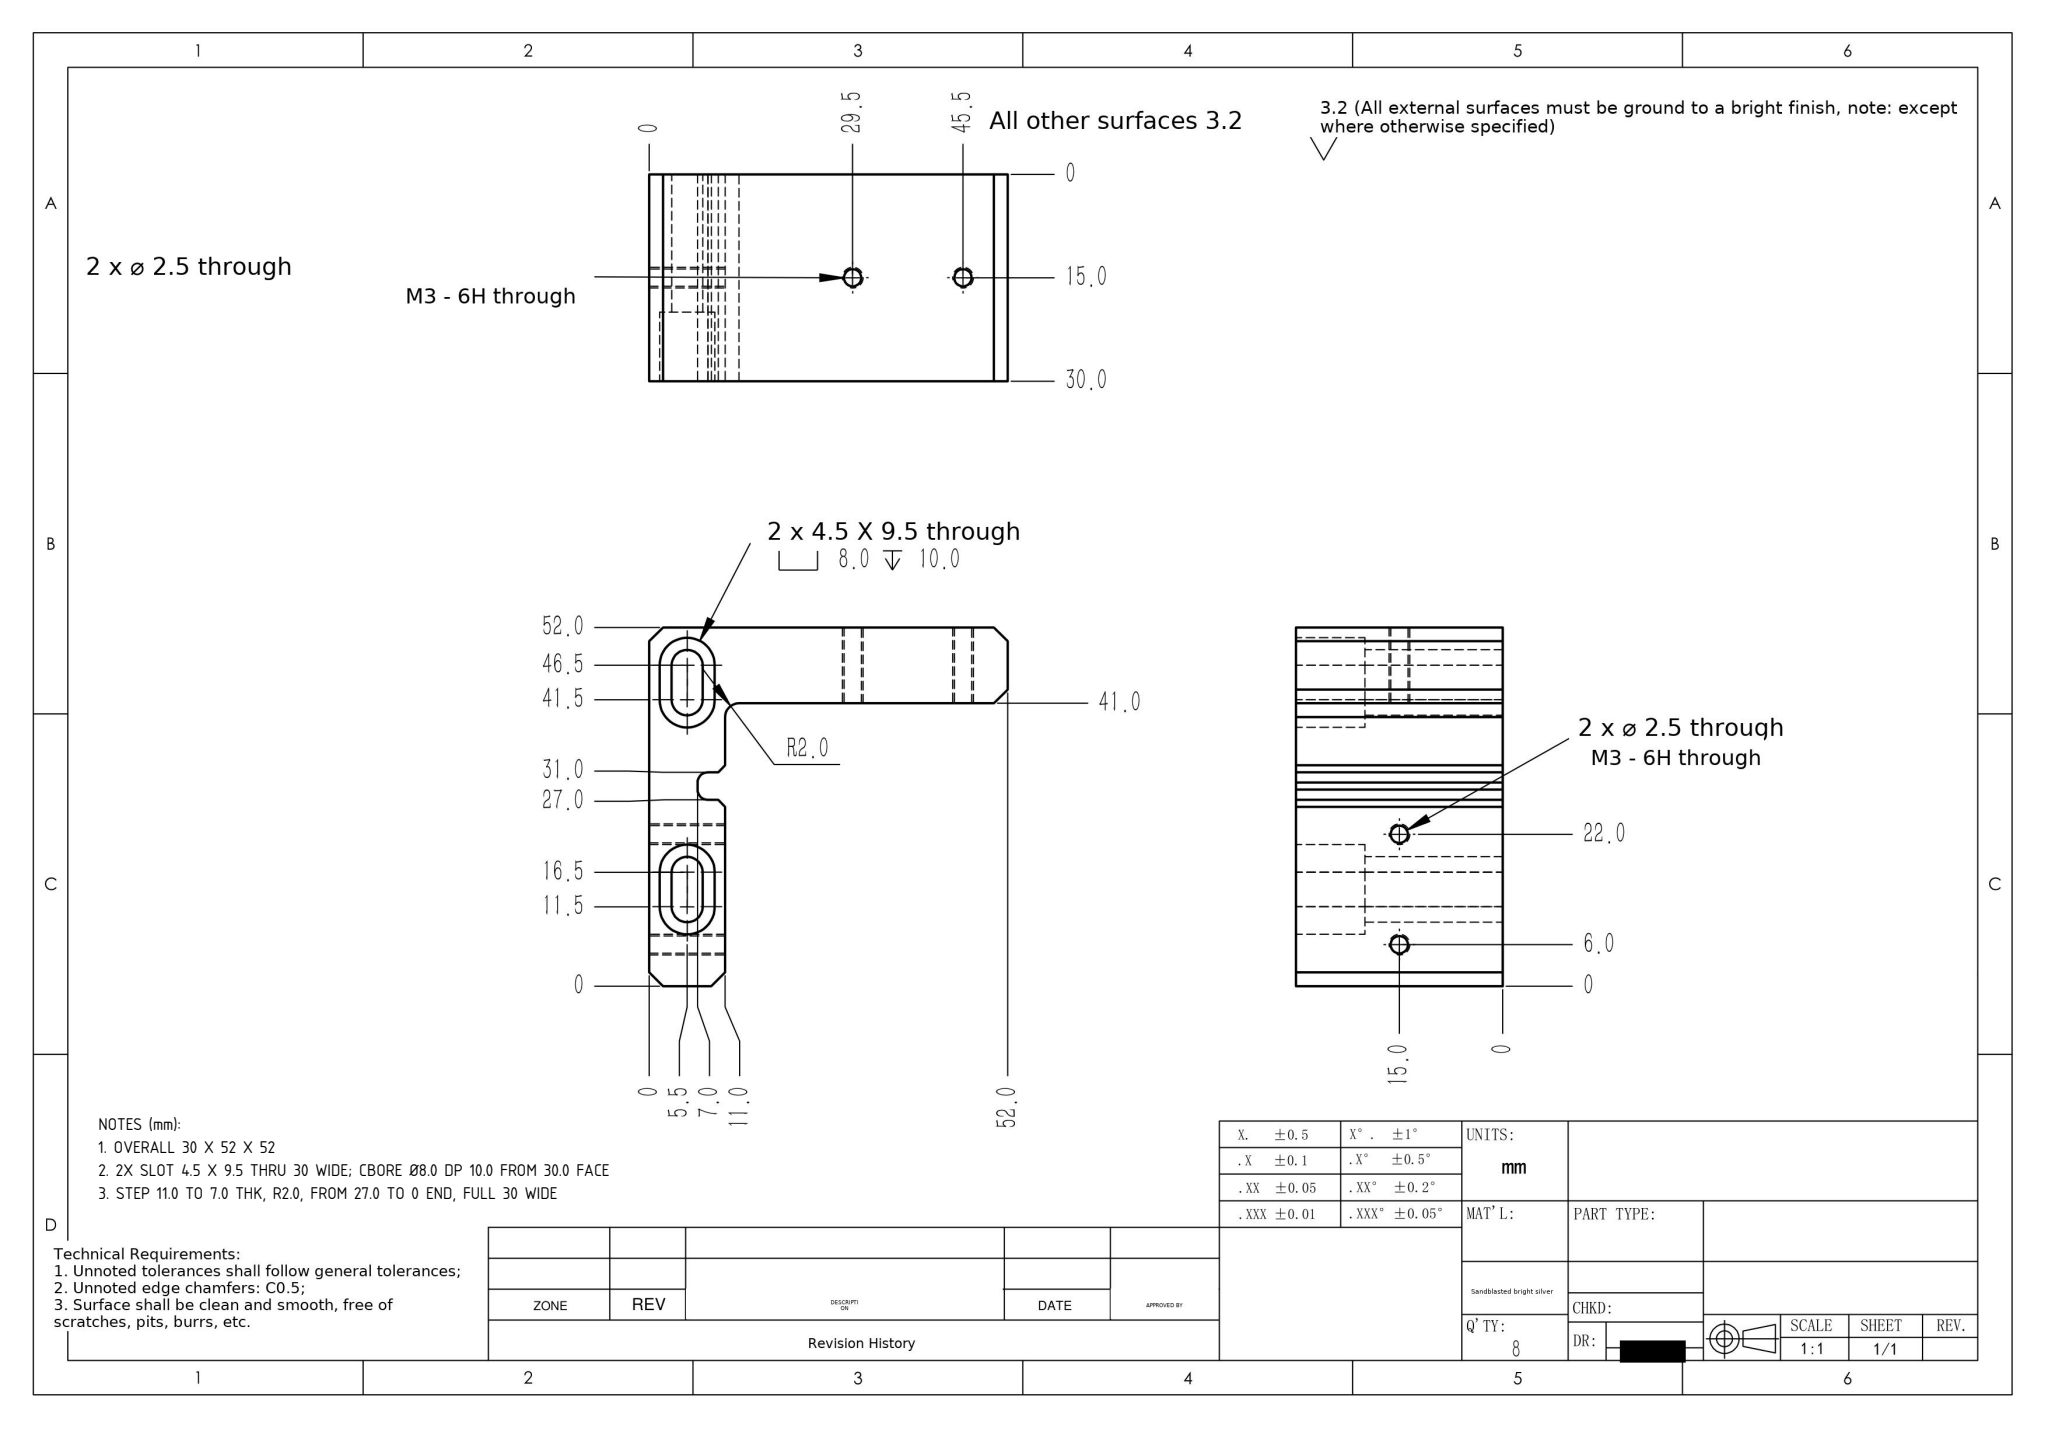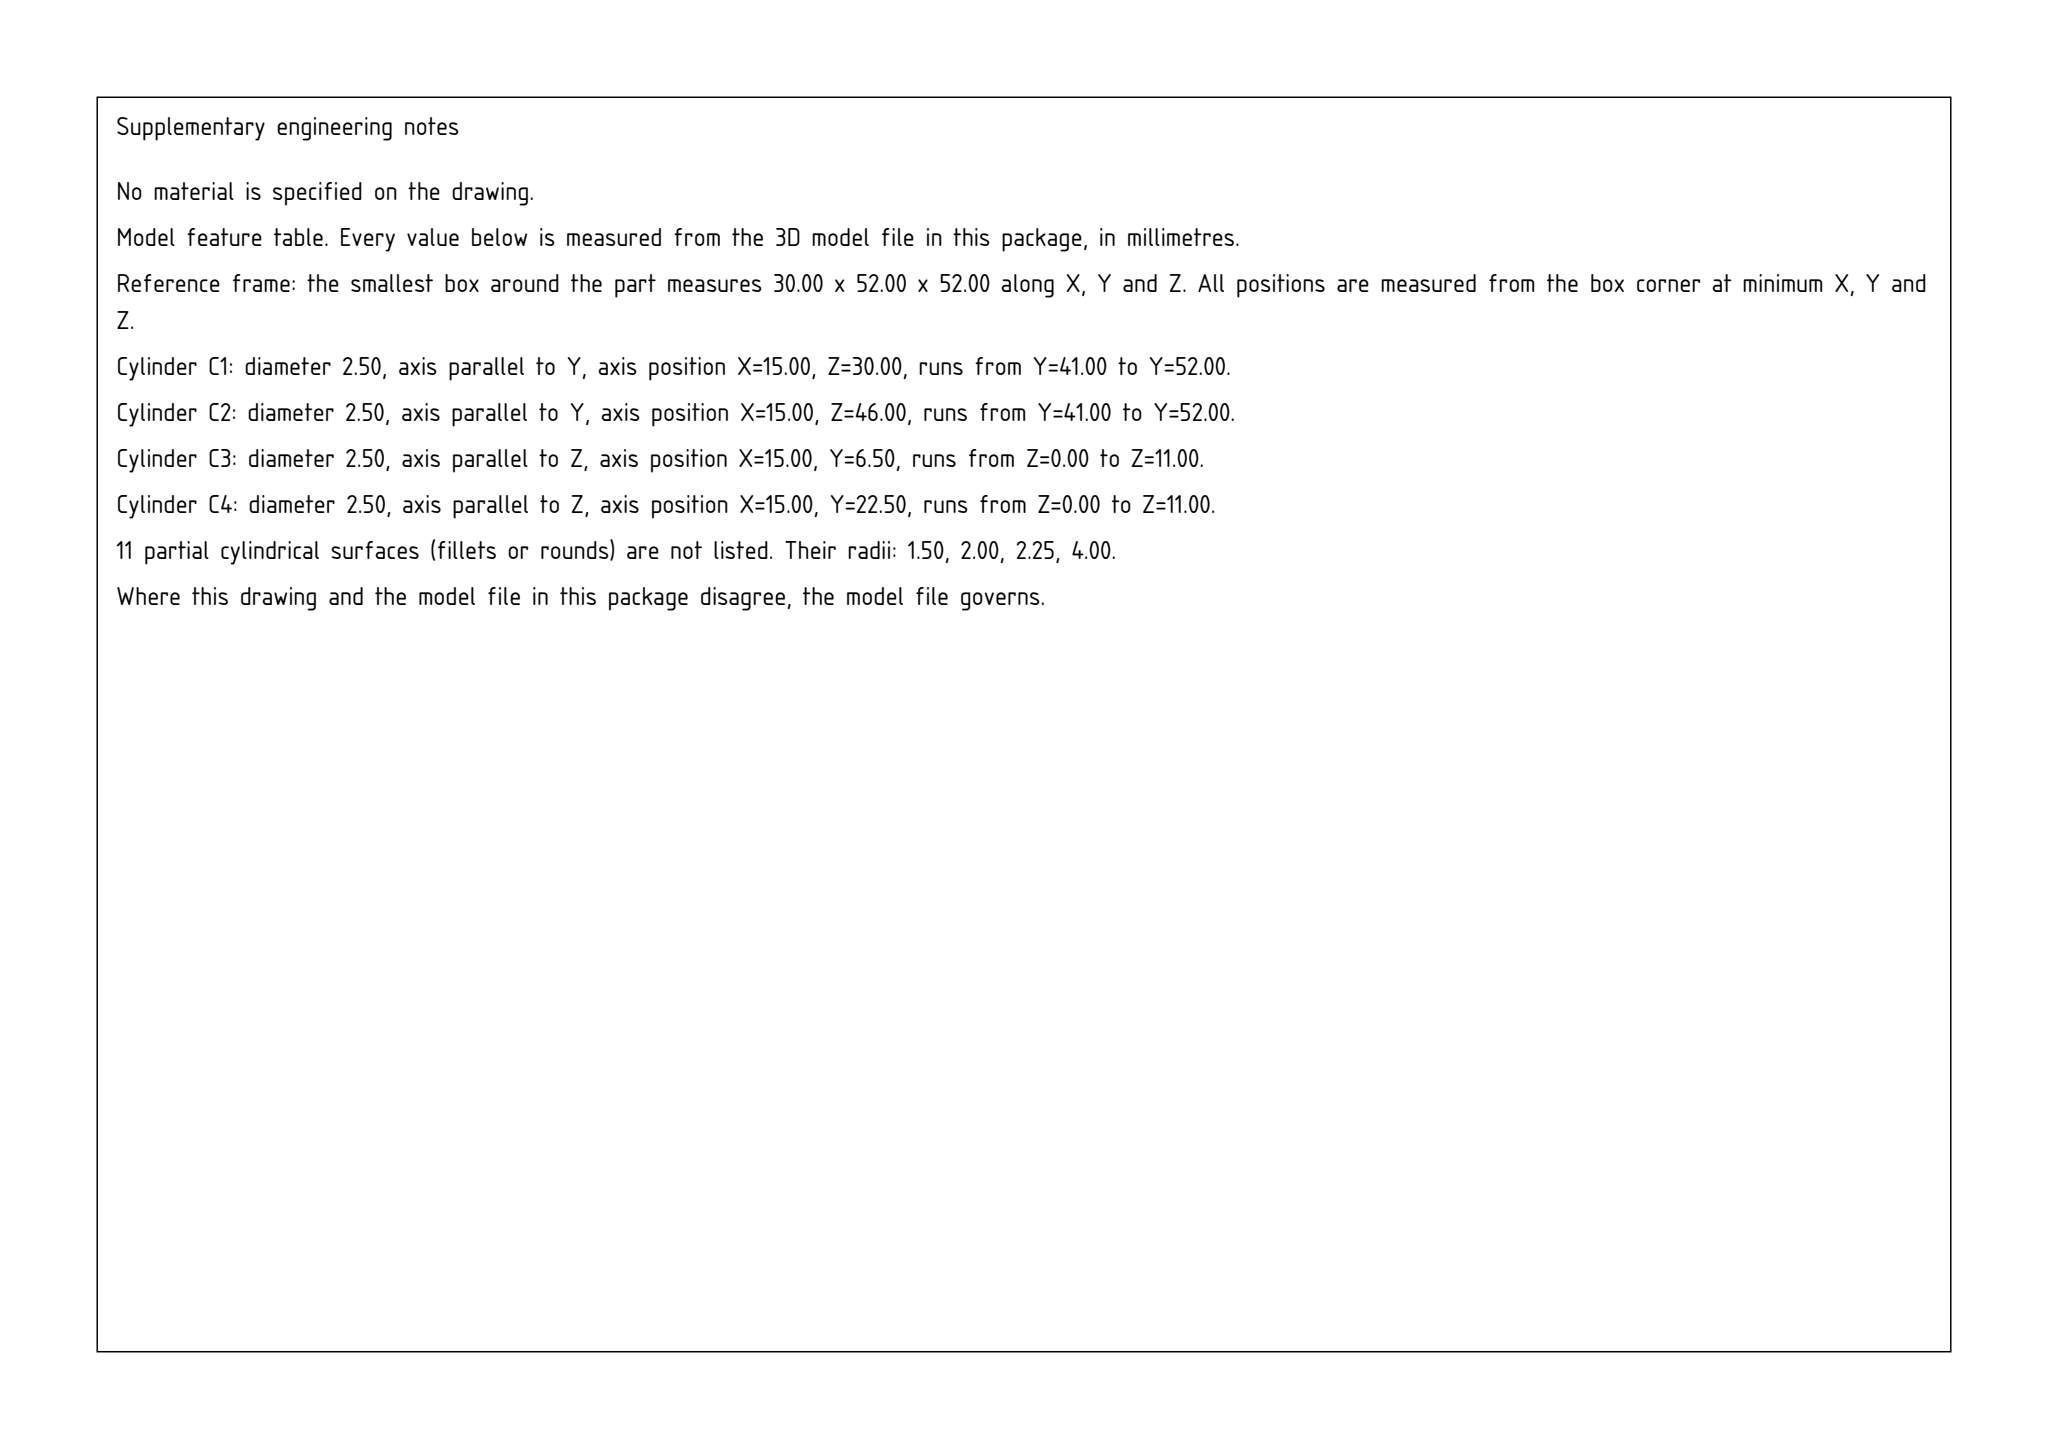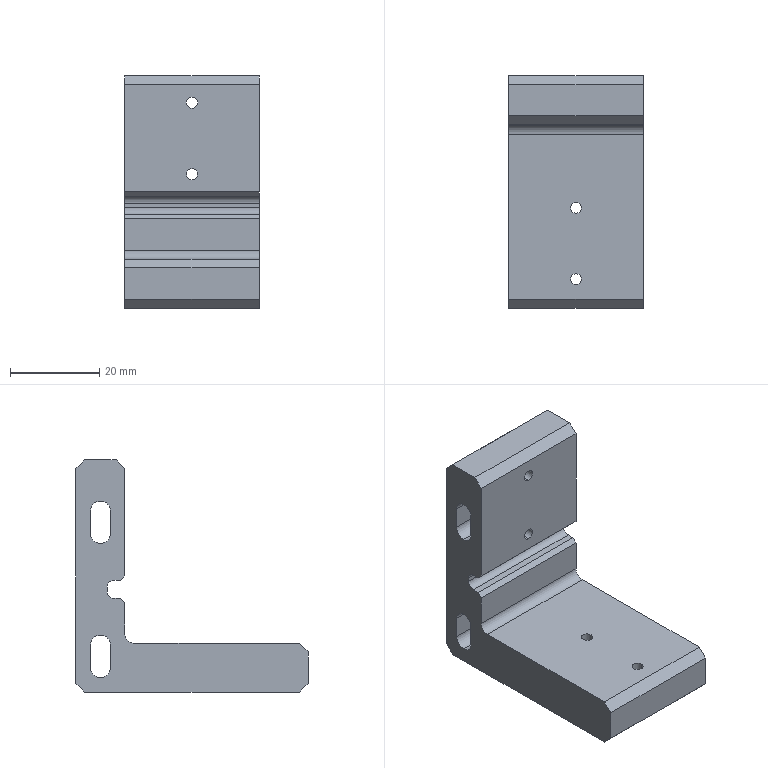Part | SolidWorks | mm | 1 solid | 52 faces | box 30 x 52 x 52 mm | volume 26377 mm3 | plane 29 | cylinder 23 | commonest cylinder face diameters 2.5 x8 8 x6 4.5 x6 3 x2 4 x1
Drawing notes:
OVERALL 30 X 52 X 52 | from the solid: bbox_xyz [30.0, 52.0, 52.0]
2X SLOT 4.5 X 9.5 THRU 30 WIDE; CBORE Ø8.0 DP 10.0 FROM 30.0 FACE | from the solid: Ø4.5 x-axis cyls L=20 @ y46.5, z5.5/10.5 & z35.5/40.5; Ø8.0 x-axis cyls L=10 same CL; x planes 0, 20 (cbore floor), 30
STEP 11.0 TO 7.0 THK, R2.0, FROM 27.0 TO 0 END, FULL 30 WIDE | from the solid: y planes 41.0 and 45.0 vs outer face y=52.0 (11.0 / 7.0 thk); z planes 21.0/25.0 = view 31.0/27.0; y=45.0 face spans x 0-30